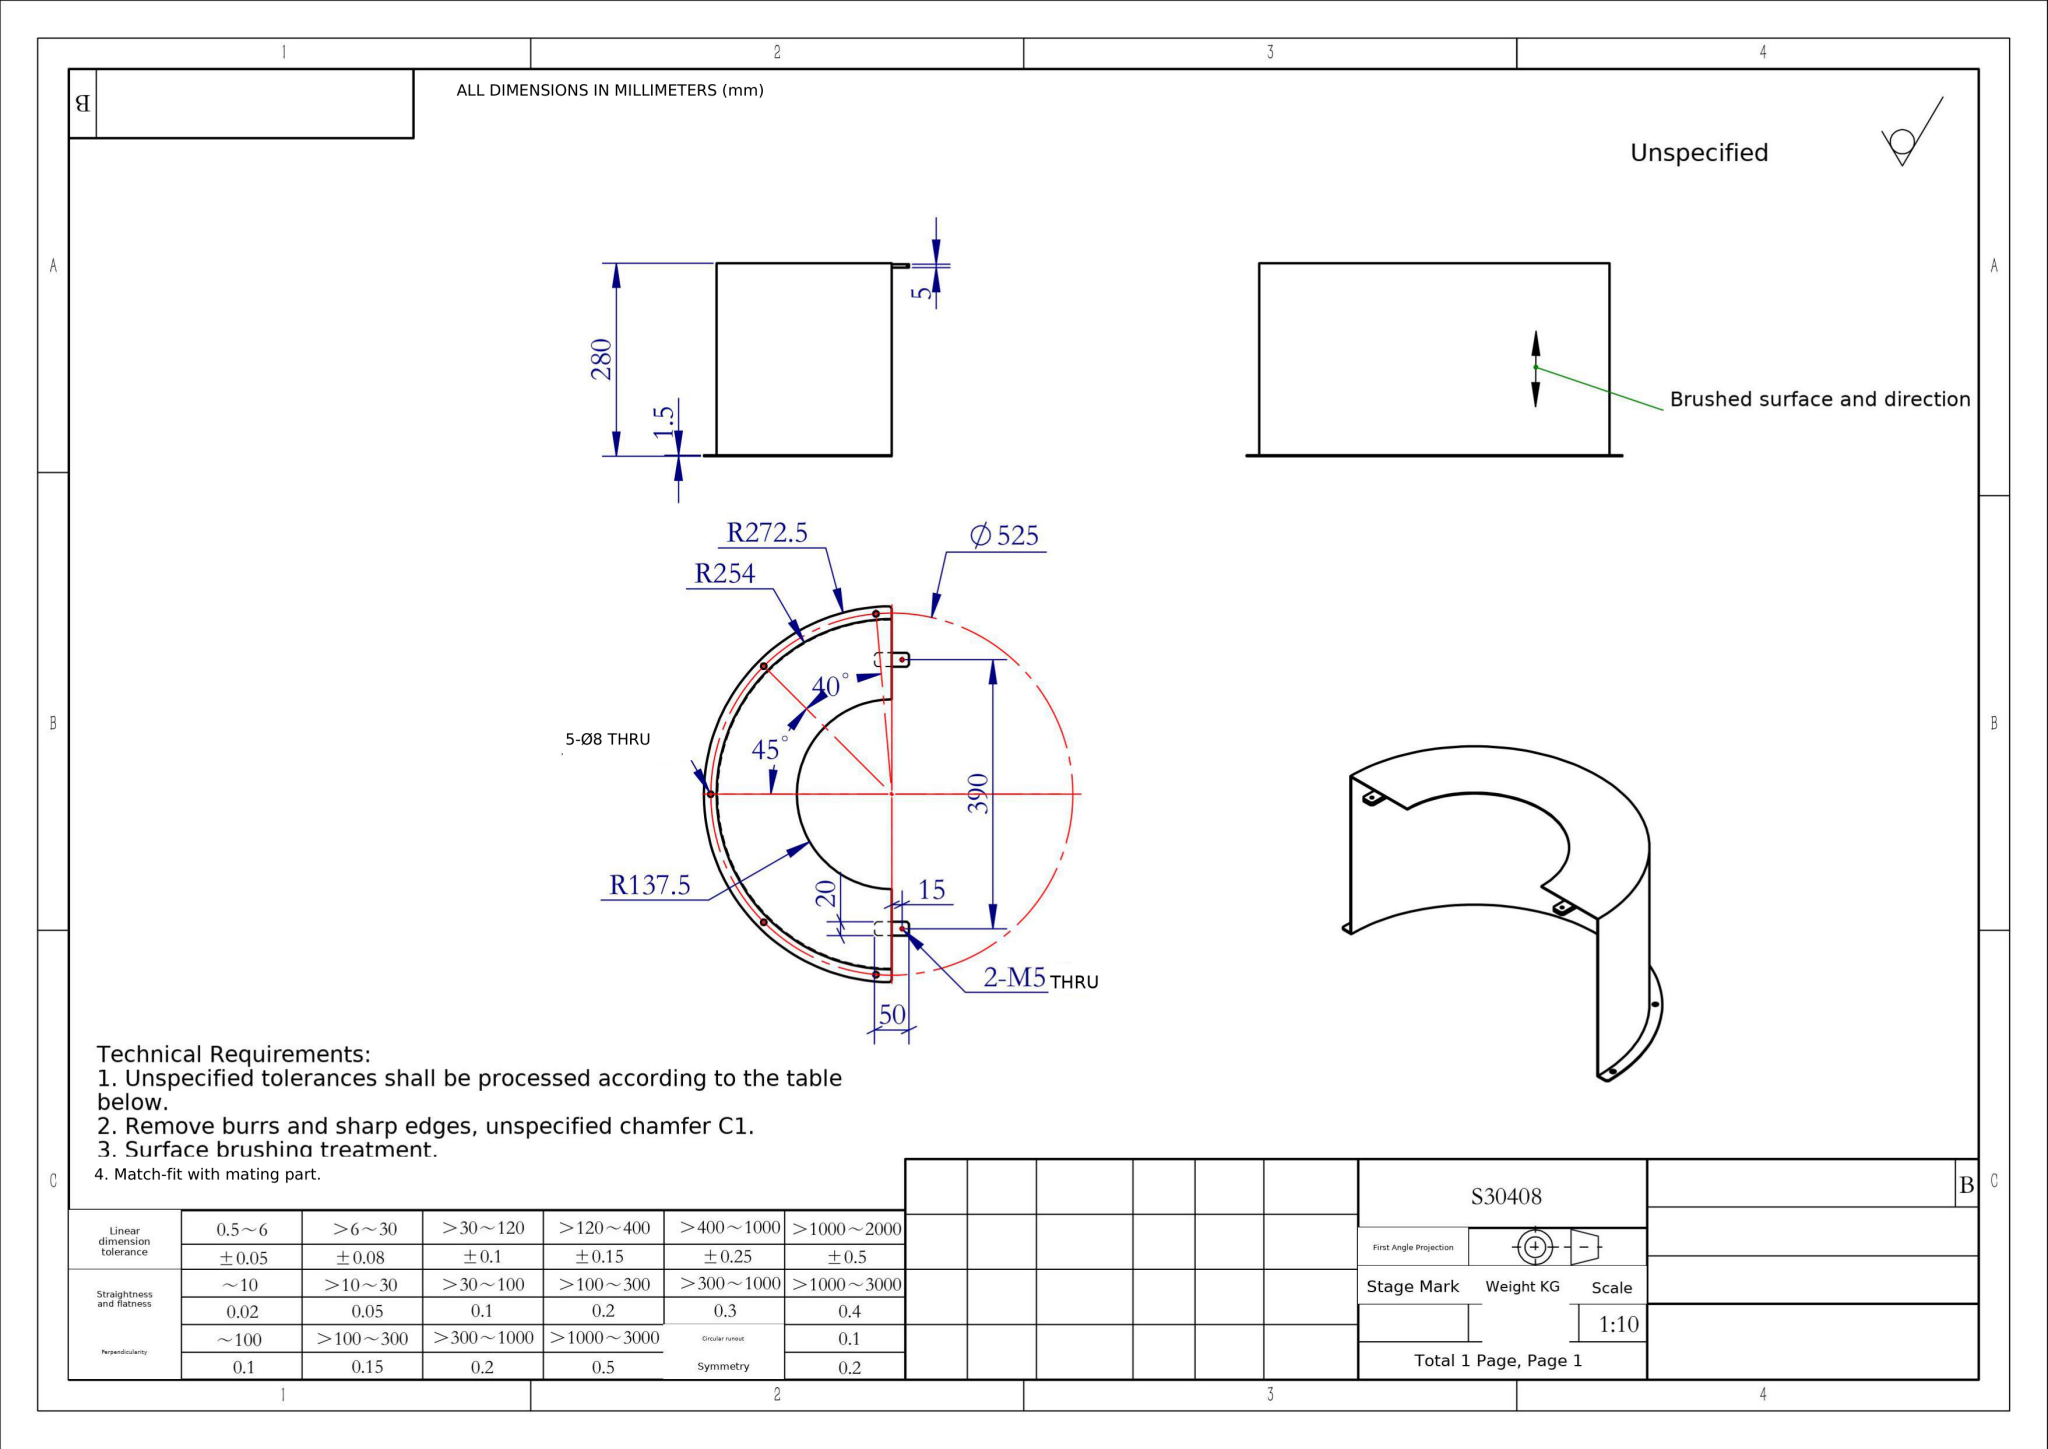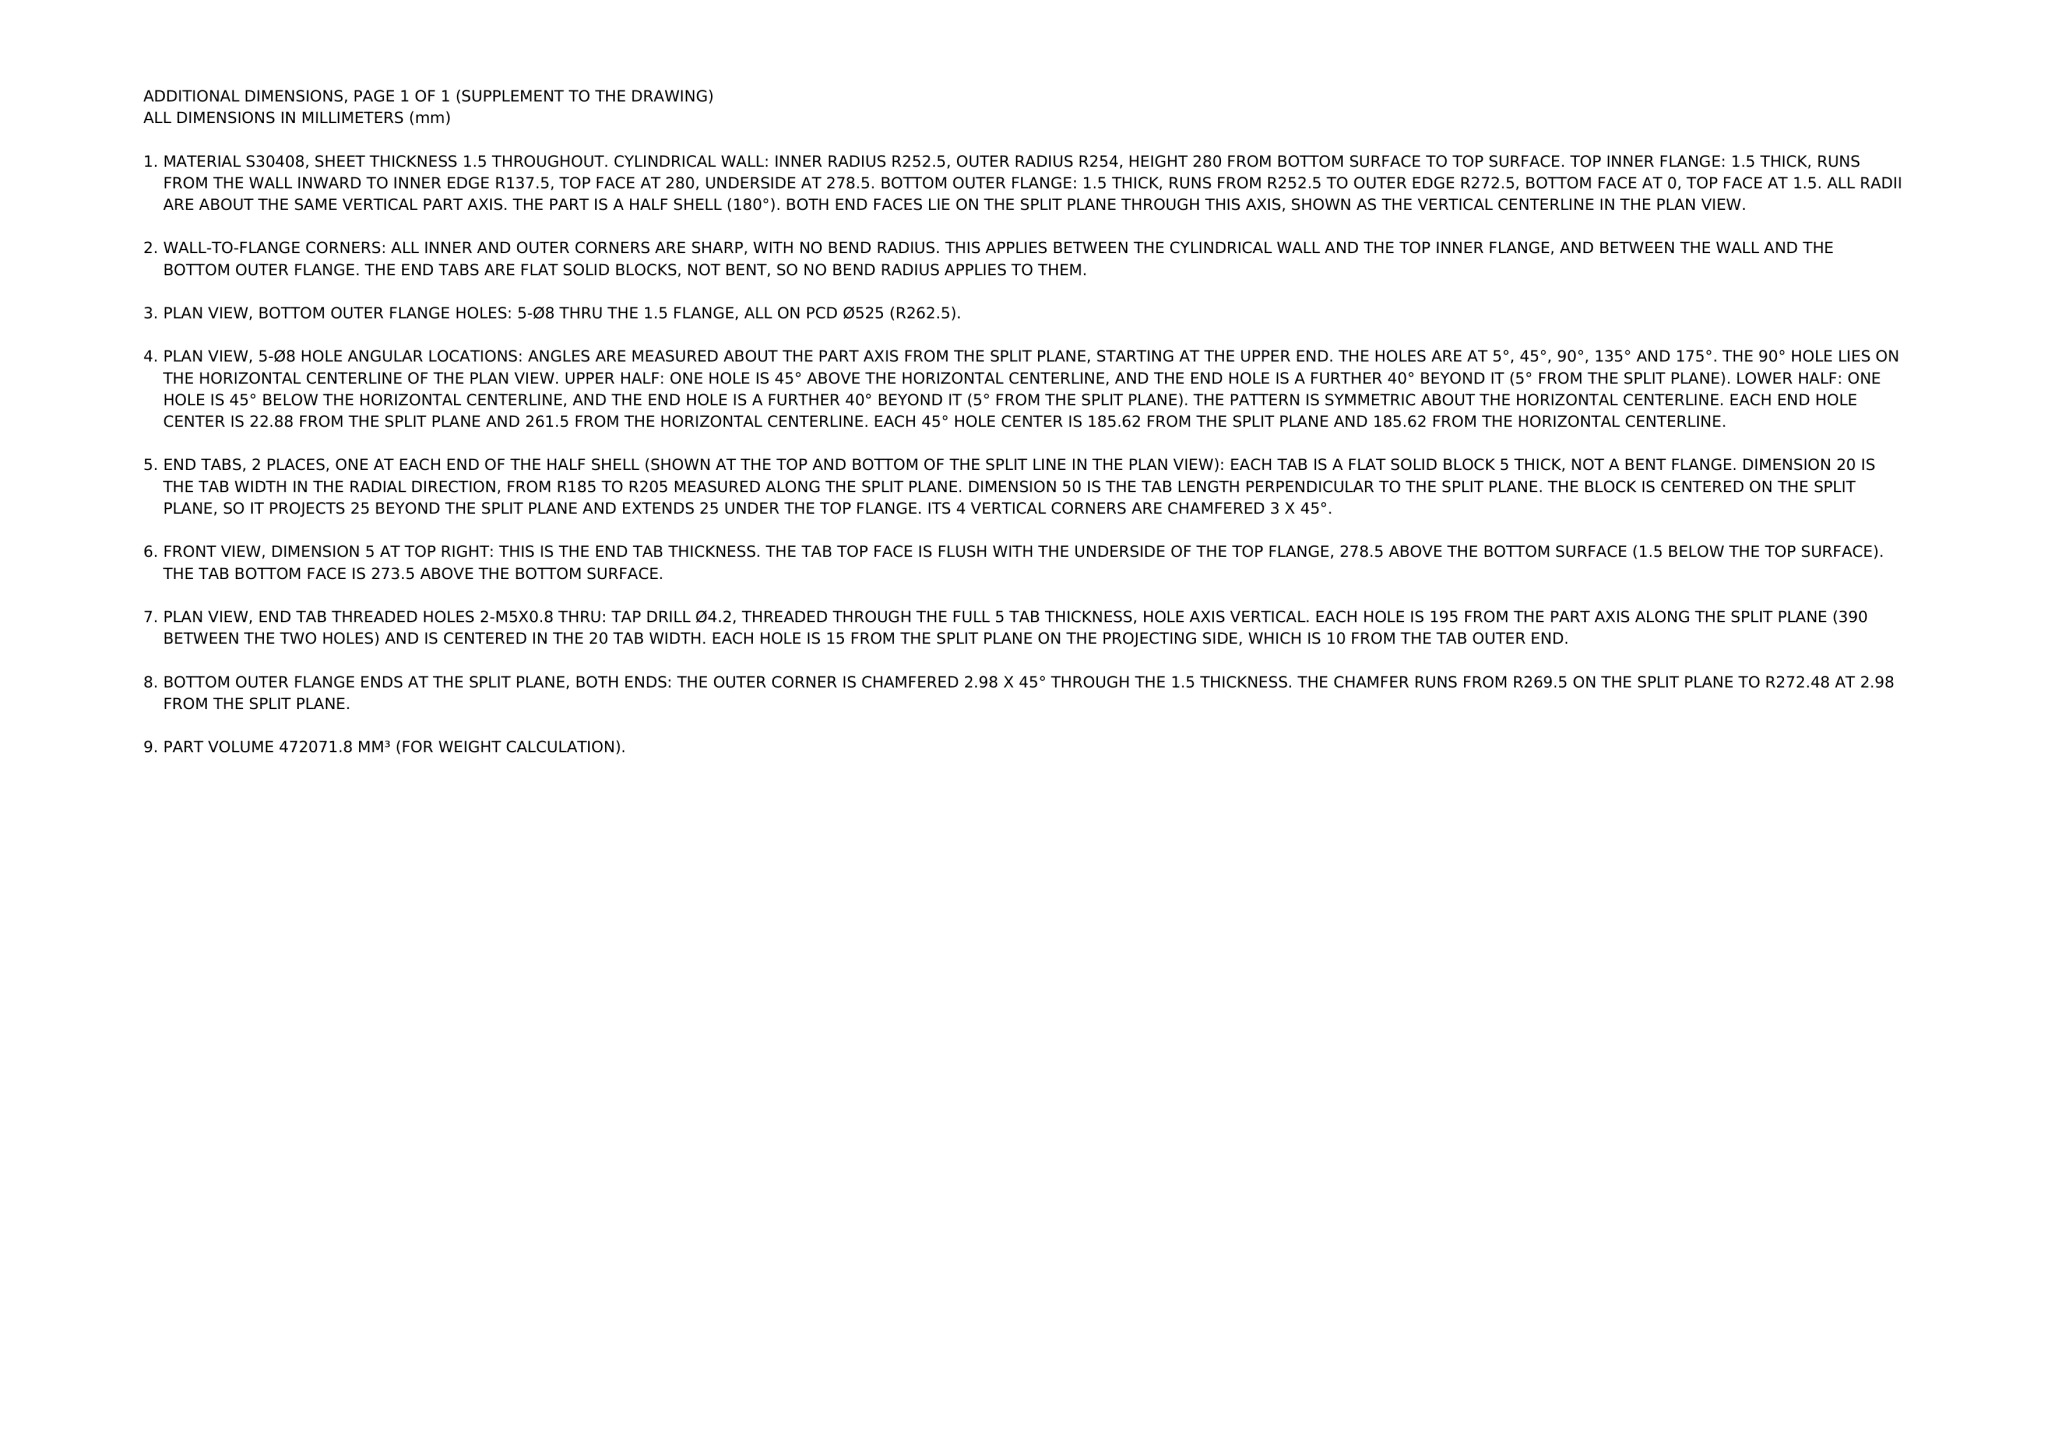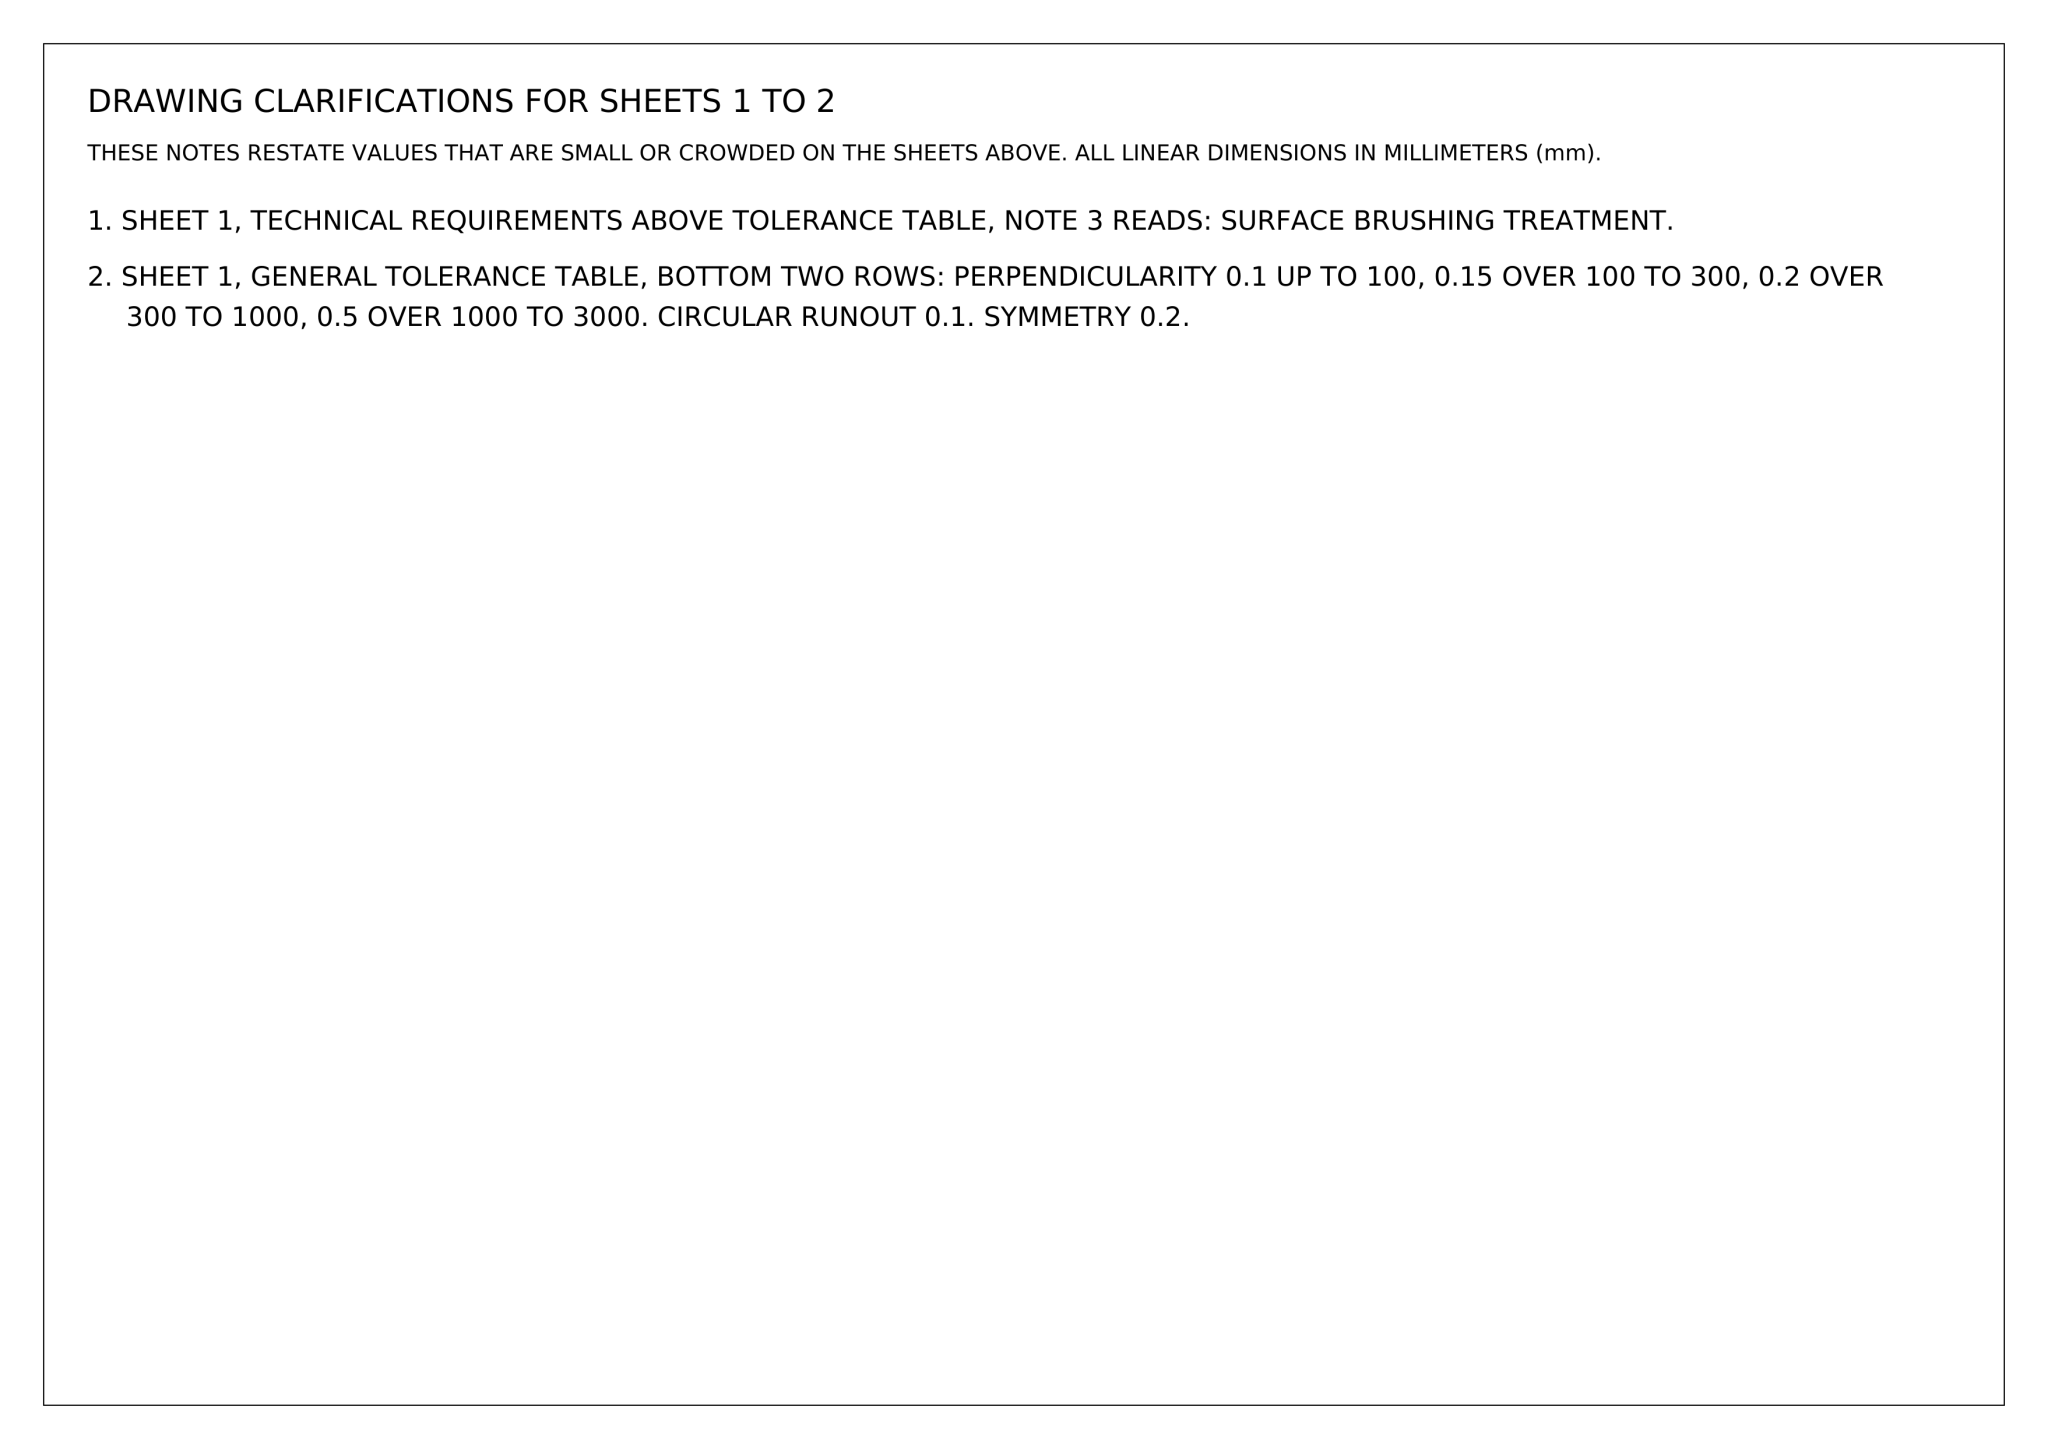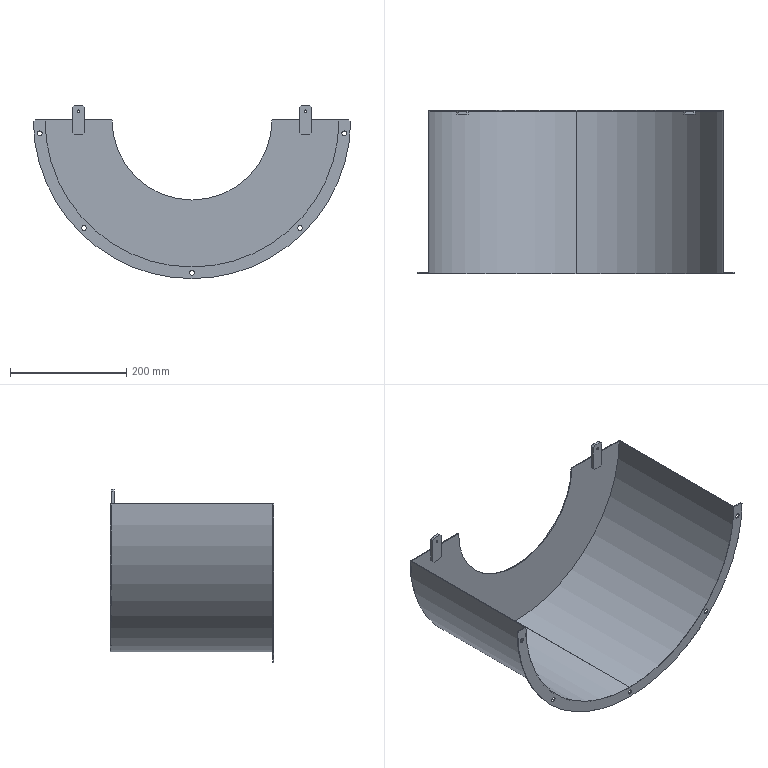Part | NX | mm | 1 solid | 49 faces | box 544.97 x 280 x 297.5 mm | volume 472072 mm3 | plane 28 | cylinder 21 | commonest cylinder face diameters 8 x10 4.2 x4 508 x2 545 x2 505 x2 275 x1